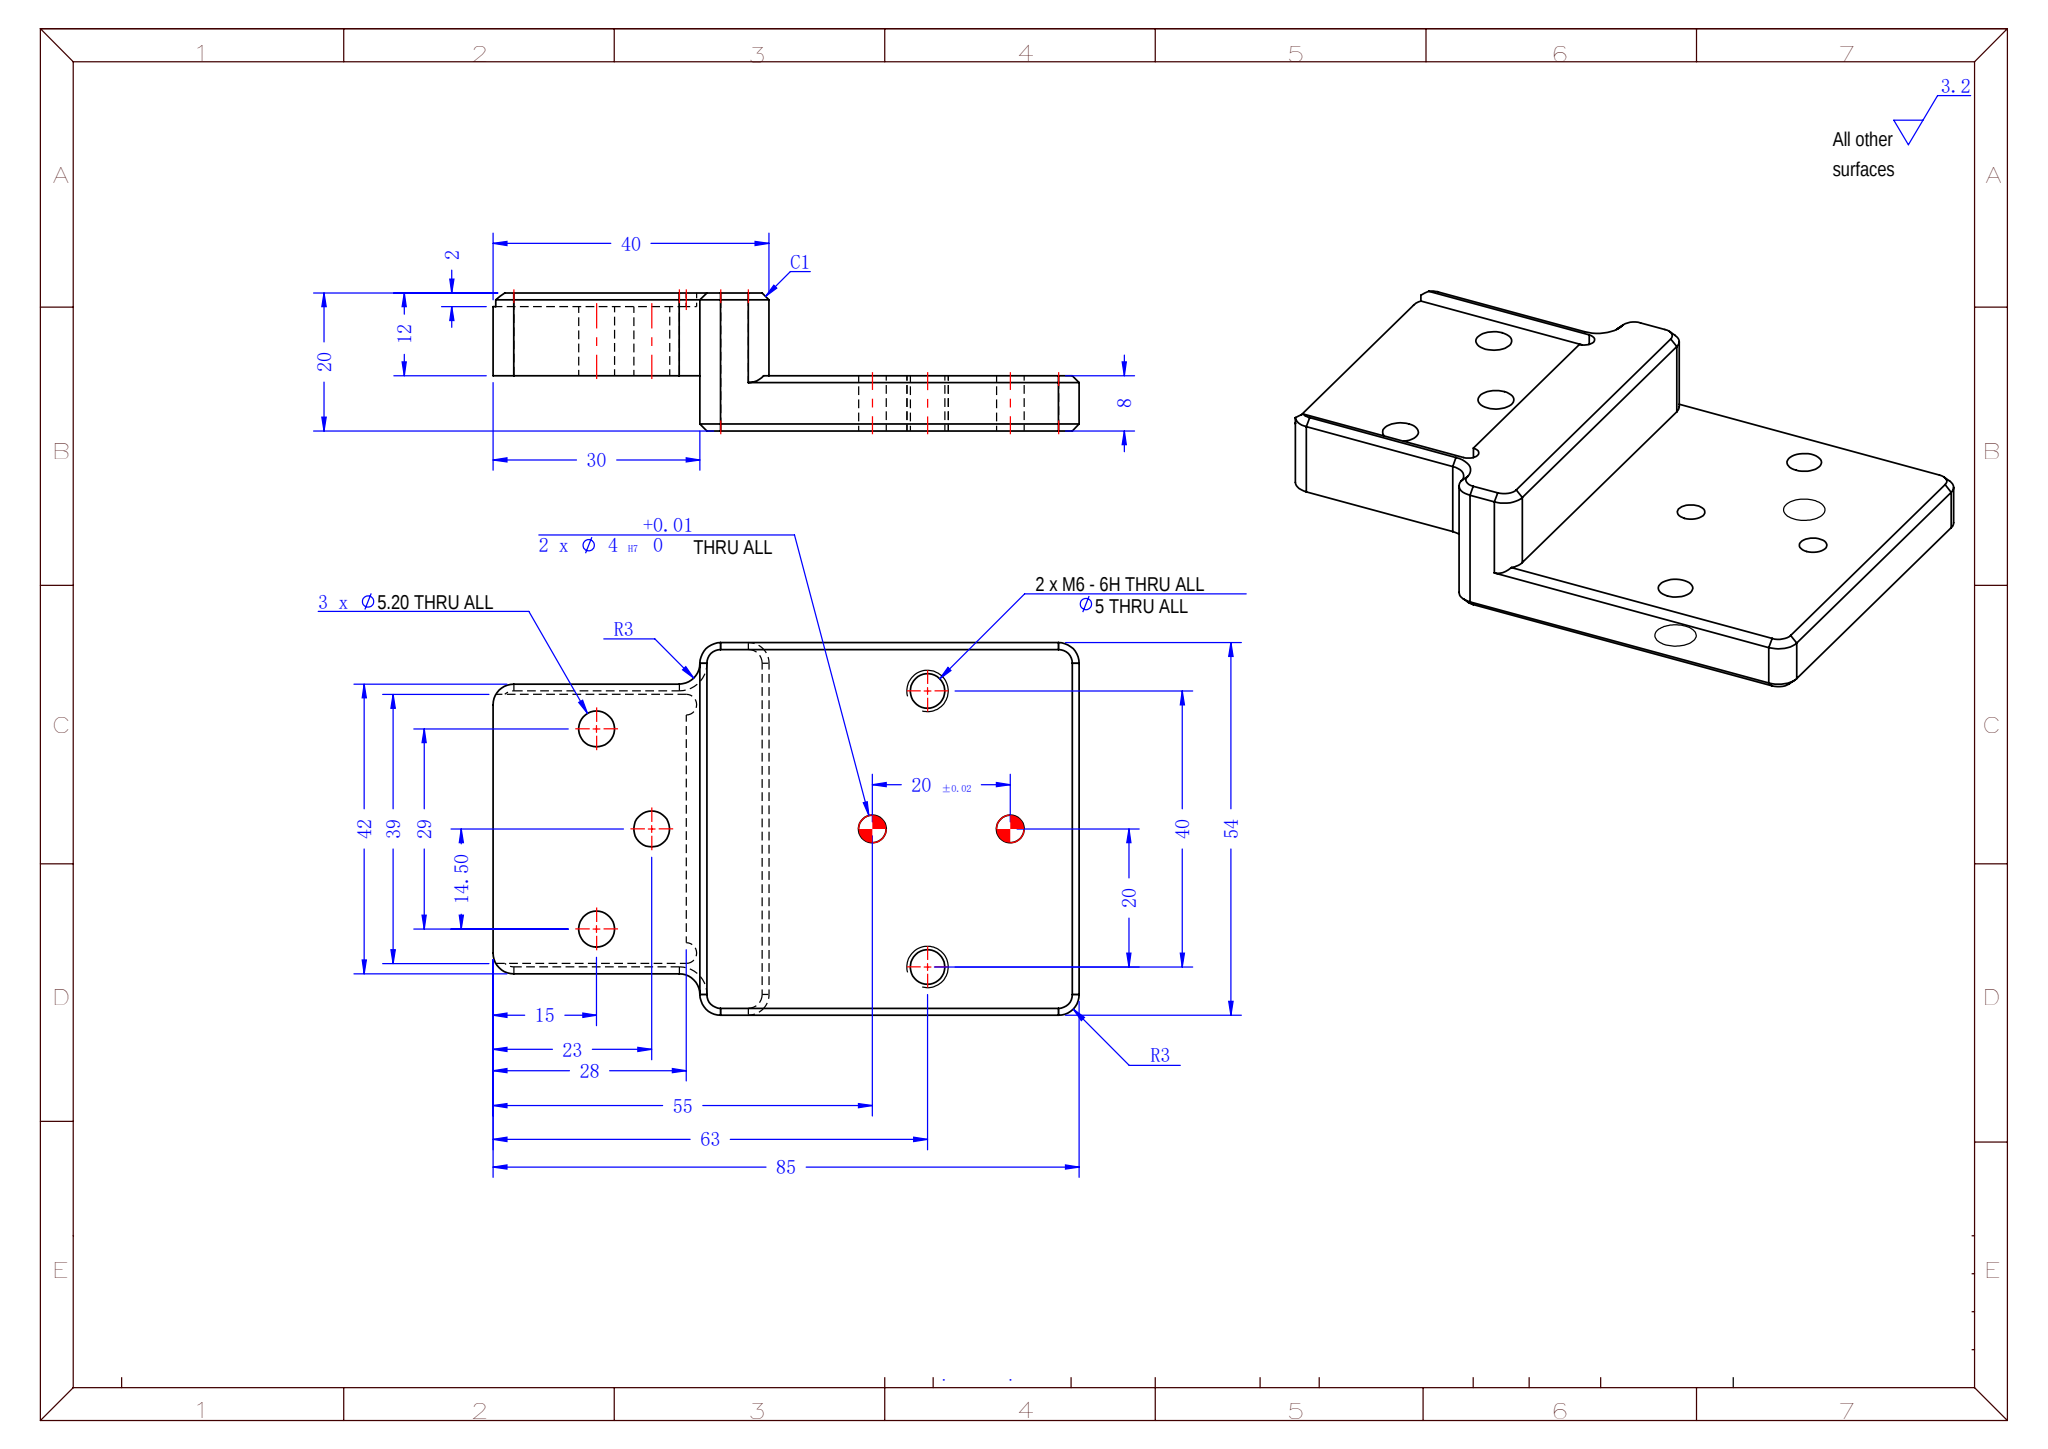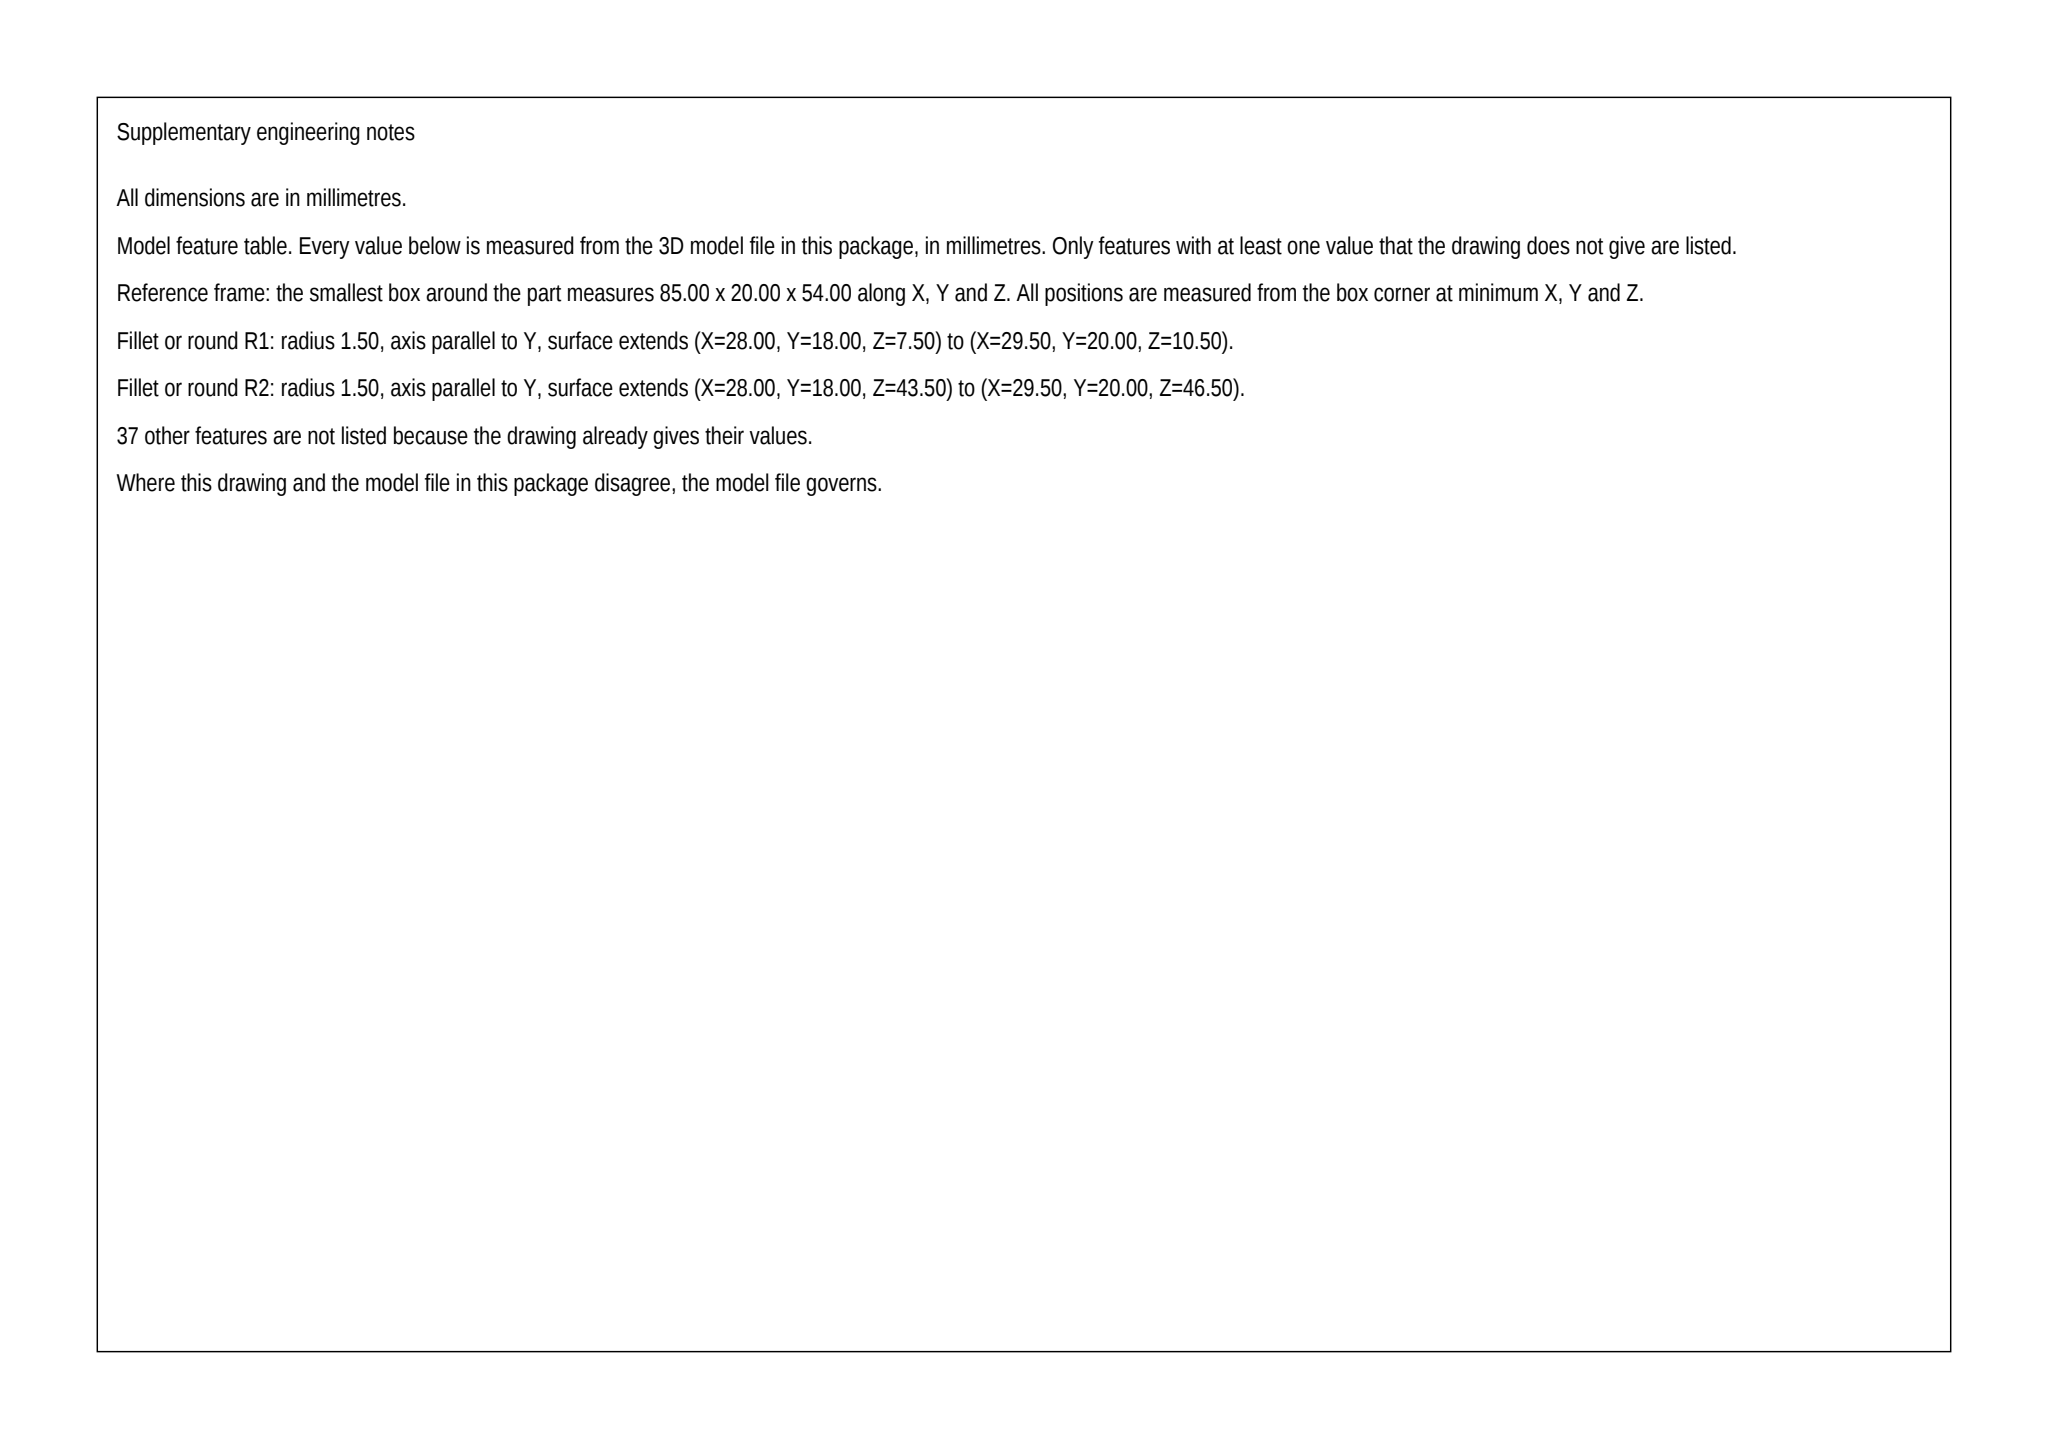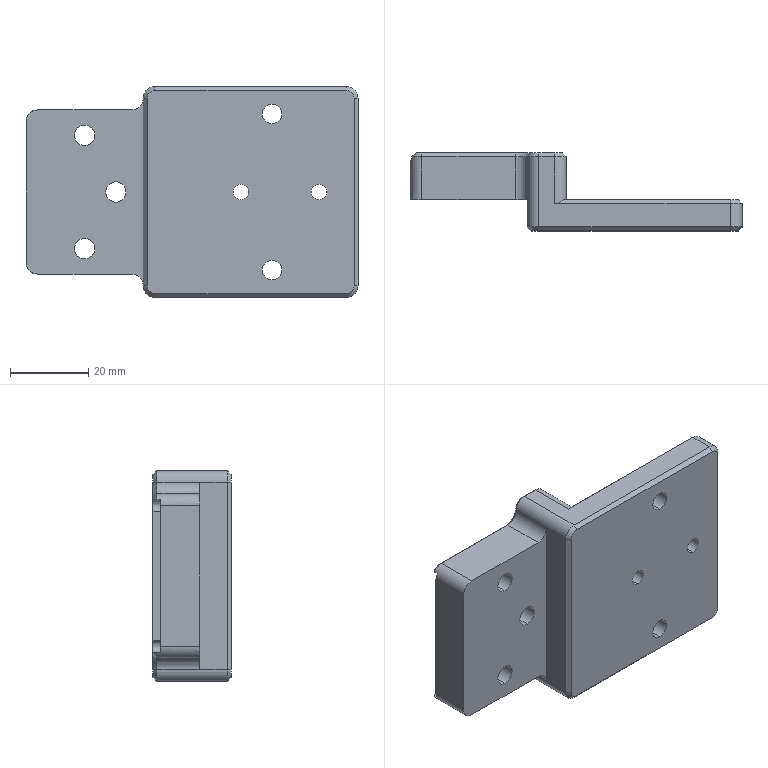Part | SolidWorks | mm | 1 solid | 68 faces | box 85 x 20 x 54 mm | volume 41610 mm3 | plane 28 | cylinder 26 | cone 14 | commonest cylinder face diameters 6 x10 5.2 x6 4 x4 5 x4 3 x2
Drawing notes:
2 HIGH PAD ON LEFT PLATE: R1.5 BOTH CORNERS AT 28 END | from the solid: Two dia 3.0 (R1.5) y-axis cyls, length 2, at x=28, z=9 & z=45; pad faces z=7.5/46.5 (39 wide), x=0..28, step top y planes 18/20
ALL HOLE ENDS 90° CHAMFER; 2 x Ø4 H7: CSK Ø8 x 90° | from the solid: cones[included_angle,ref_dia]: [90.0,4.0]x12 and [90.0,8.0]x2; dia 4.0 holes at x=55 & x=75, z=27 (2 x 4 H7)
R3 TYP AT 2 CORNERS, LEFT (X=0) END OF RAISED PLATE - TOP VIEW | from the solid: Vertical cyl dia 6.0 (R3), axis Y, at x=3 z=9 and x=3 z=45, tangent to face x=0 and to z=6 / z=48 edges of the raised left plate
ALL HOLE ENDS: CHAMFER 90° INCLUDED TO Ø4 REF (CHAMFER LEG = (Ø4 - HOLE Ø)/2), 12 PLACES, BOTH FACES | from the solid: cones[included_angle,ref_dia] = [90.0, 4.0, 12]
2 × Ø4 H7 HOLES (Y AXIS AT X=55 AND X=75, Z=27 FROM BBOX MIN CORNER): CSK Ø8 × 90°, CSK DEPTH 2.0 ((Ø8-Ø4)/2) | from the solid: cones[included_angle,ref_dia] = [90.0, 8.0, 2] with cylinders [4.0,'y',[55.0,null,27.0],8.0] and [4.0,'y',[75.0,null,27.0],8.0]